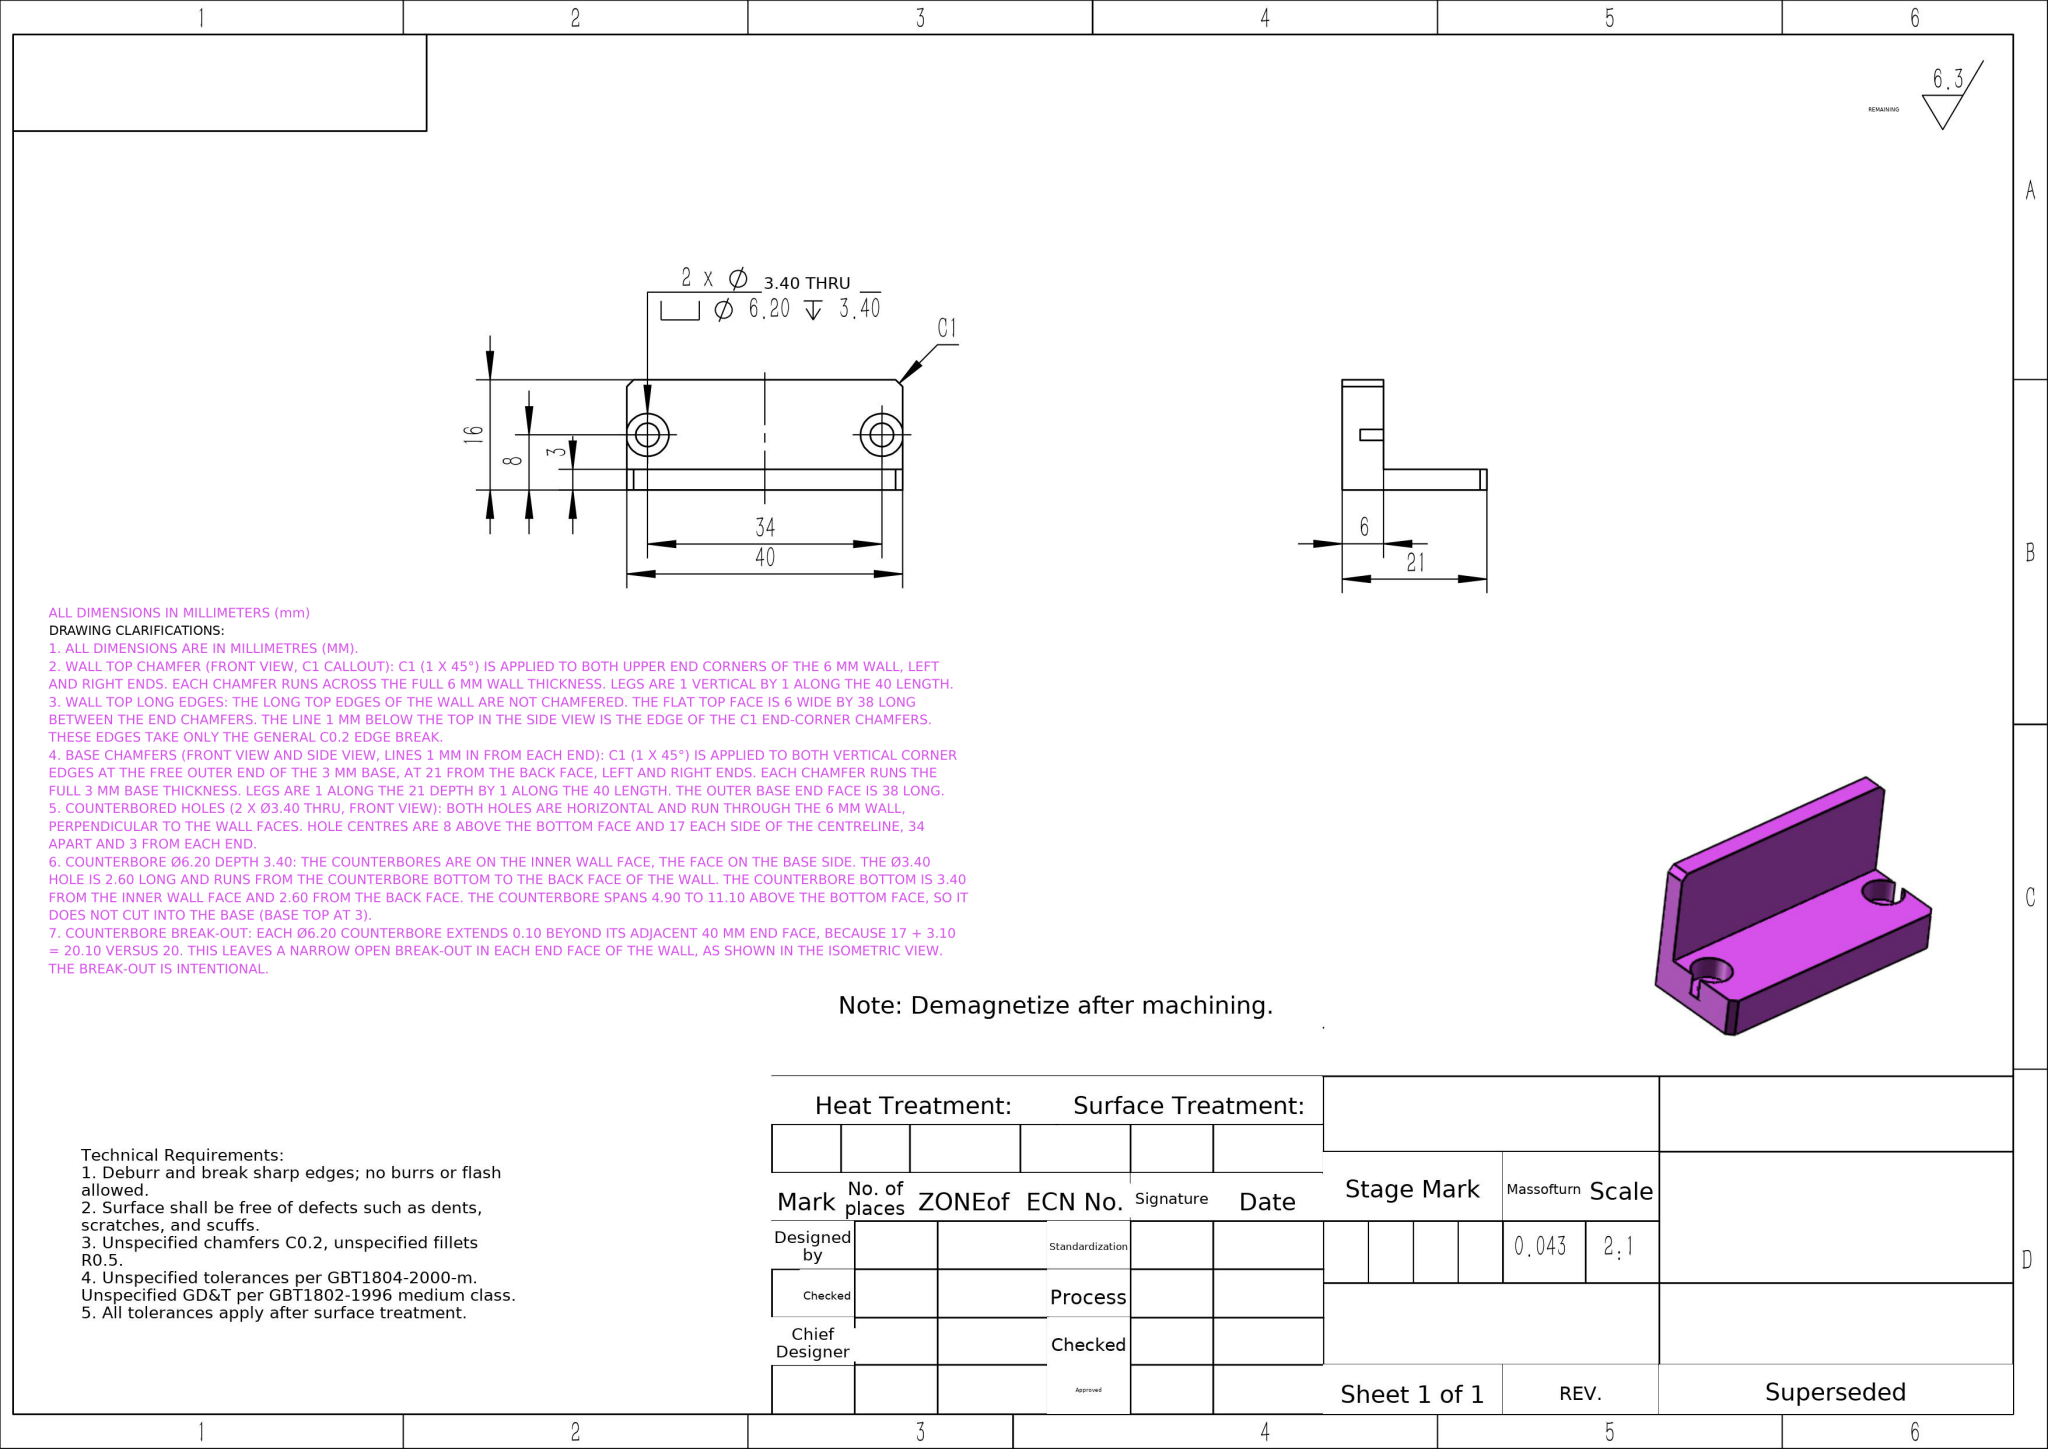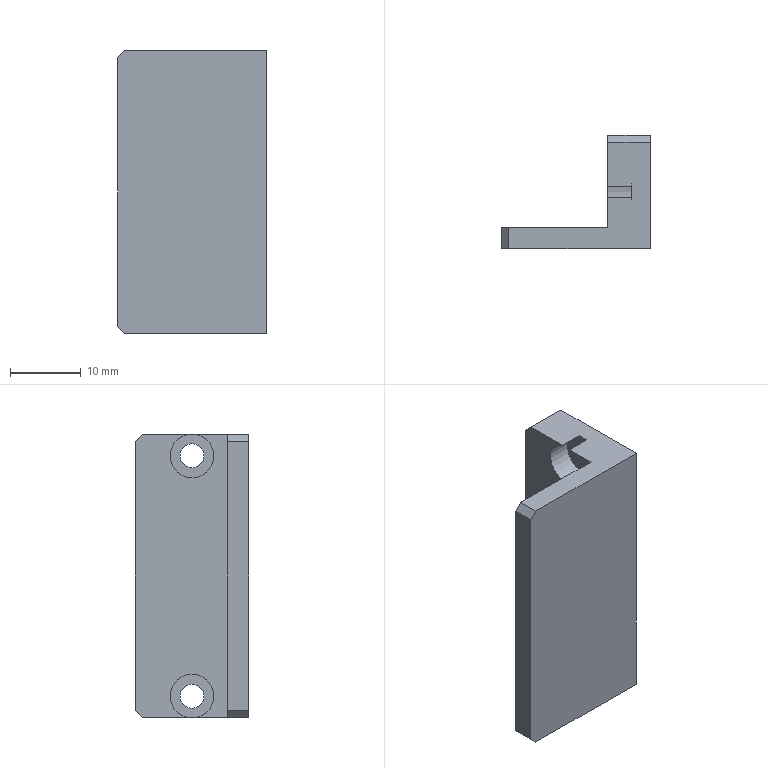Part | NX | mm | V-Notched Two-Bore Vertical Block | 1 solid | 21 faces | box 21 x 16 x 40 mm | volume 5379 mm3 | plane 14 | cylinder 7 | commonest cylinder face diameters 3.4 x4 6.2 x3
STEP:
#1=COLOUR_RGB('',0.6471,0.6196,0.5882);
#2=FILL_AREA_STYLE_COLOUR('',#1);
#3=FILL_AREA_STYLE('',(#2));
#4=SURFACE_STYLE_FILL_AREA(#3);
#5=SURFACE_SIDE_STYLE('',(#4));
#6=SURFACE_STYLE_USAGE(.BOTH.,#5);
#7=PRESENTATION_STYLE_ASSIGNMENT((#6));
#8=CARTESIAN_POINT('',(-2.6,-8.,-13.9));
#9=VERTEX_POINT('',#8);
#10=CARTESIAN_POINT('',(-2.6,-7.219,-20.));
#11=VERTEX_POINT('',#10);
#12=CARTESIAN_POINT('',(-2.6,-8.,-17.));
#13=DIRECTION('',(-1.,0.,0.));
#14=DIRECTION('',(0.,0.,1.));
#15=AXIS2_PLACEMENT_3D('',#12,#13,#14);
#16=CIRCLE('',#15,3.1);
#17=EDGE_CURVE('',#9,#11,#16,.T.);
#18=ORIENTED_EDGE('',*,*,#17,.F.);
#19=CARTESIAN_POINT('',(-6.,-8.,-13.9));
#20=VERTEX_POINT('',#19);
#21=CARTESIAN_POINT('',(-6.,-8.,-13.9));
#22=DIRECTION('',(-1.,0.,0.));
#23=VECTOR('',#22,1000.);
#24=LINE('',#21,#23);
#25=EDGE_CURVE('',#9,#20,#24,.T.);
#26=ORIENTED_EDGE('',*,*,#25,.T.);
#27=CARTESIAN_POINT('',(-6.,-7.219,-20.));
#28=VERTEX_POINT('',#27);
#29=CARTESIAN_POINT('',(-6.,-8.,-17.));
#30=DIRECTION('',(-1.,0.,0.));
#31=DIRECTION('',(0.,0.,1.));
#32=AXIS2_PLACEMENT_3D('',#29,#30,#31);
#33=CIRCLE('',#32,3.1);
#34=EDGE_CURVE('',#20,#28,#33,.T.);
#35=ORIENTED_EDGE('',*,*,#34,.T.);
#36=CARTESIAN_POINT('',(-6.,-7.219,-20.));
#37=DIRECTION('',(1.,0.,0.));
#38=VECTOR('',#37,1000.);
#39=LINE('',#36,#38);
#40=EDGE_CURVE('',#28,#11,#39,.T.);
#41=ORIENTED_EDGE('',*,*,#40,.T.);
#42=EDGE_LOOP('',(#18,#26,#35,#41));
#43=FACE_OUTER_BOUND('',#42,.T.);
#44=CARTESIAN_POINT('',(-6.,-8.,-17.));
#45=DIRECTION('',(-1.,0.,0.));
#46=DIRECTION('',(0.,0.,1.));
#47=AXIS2_PLACEMENT_3D('',#44,#45,#46);
#48=CYLINDRICAL_SURFACE('',#47,3.1);
#49=ADVANCED_FACE('',(#43),#48,.F.);
#50=CARTESIAN_POINT('',(0.,-8.,-18.7));
#51=VERTEX_POINT('',#50);
#52=CARTESIAN_POINT('',(0.,-8.,-15.3));
#53=VERTEX_POINT('',#52);
#54=CARTESIAN_POINT('',(0.,-8.,-17.));
#55=DIRECTION('',(-1.,-0.,0.));
#56=DIRECTION('',(0.,-1.,0.));
#57=AXIS2_PLACEMENT_3D('',#54,#55,#56);
#58=CIRCLE('',#57,1.7);
#59=EDGE_CURVE('',#51,#53,#58,.T.);
#60=ORIENTED_EDGE('',*,*,#59,.F.);
#61=CARTESIAN_POINT('',(-2.6,-8.,-18.7));
#62=VERTEX_POINT('',#61);
#63=CARTESIAN_POINT('',(-6.,-8.,-18.7));
#64=DIRECTION('',(-1.,0.,0.));
#65=VECTOR('',#64,1000.);
#66=LINE('',#63,#65);
#67=EDGE_CURVE('',#51,#62,#66,.T.);
#68=ORIENTED_EDGE('',*,*,#67,.T.);
#69=CARTESIAN_POINT('',(-2.6,-8.,-15.3));
#70=VERTEX_POINT('',#69);
#71=CARTESIAN_POINT('',(-2.6,-8.,-17.));
#72=DIRECTION('',(-1.,0.,0.));
#73=DIRECTION('',(0.,0.,1.));
#74=AXIS2_PLACEMENT_3D('',#71,#72,#73);
#75=CIRCLE('',#74,1.7);
#76=EDGE_CURVE('',#62,#70,#75,.T.);
#77=ORIENTED_EDGE('',*,*,#76,.T.);
#78=CARTESIAN_POINT('',(-6.,-8.,-15.3));
#79=DIRECTION('',(-1.,0.,0.));
#80=VECTOR('',#79,1000.);
#81=LINE('',#78,#80);
#82=EDGE_CURVE('',#53,#70,#81,.T.);
#83=ORIENTED_EDGE('',*,*,#82,.F.);
#84=EDGE_LOOP('',(#60,#68,#77,#83));
#85=FACE_OUTER_BOUND('',#84,.T.);
#86=CARTESIAN_POINT('',(-6.,-8.,-17.));
#87=DIRECTION('',(-1.,0.,0.));
#88=DIRECTION('',(0.,0.,1.));
#89=AXIS2_PLACEMENT_3D('',#86,#87,#88);
#90=CYLINDRICAL_SURFACE('',#89,1.7);
#91=ADVANCED_FACE('',(#85),#90,.F.);
#92=CARTESIAN_POINT('',(0.,-8.,15.3));
#93=VERTEX_POINT('',#92);
#94=CARTESIAN_POINT('',(0.,-8.,18.7));
#95=VERTEX_POINT('',#94);
#96=CARTESIAN_POINT('',(0.,-8.,17.));
#97=DIRECTION('',(-1.,-0.,0.));
#98=DIRECTION('',(0.,-1.,0.));
#99=AXIS2_PLACEMENT_3D('',#96,#97,#98);
#100=CIRCLE('',#99,1.7);
#101=EDGE_CURVE('',#93,#95,#100,.T.);
#102=ORIENTED_EDGE('',*,*,#101,.F.);
#103=CARTESIAN_POINT('',(-2.6,-8.,15.3));
#104=VERTEX_POINT('',#103);
#105=CARTESIAN_POINT('',(-6.,-8.,15.3));
#106=DIRECTION('',(-1.,0.,0.));
#107=VECTOR('',#106,1000.);
#108=LINE('',#105,#107);
#109=EDGE_CURVE('',#93,#104,#108,.T.);
#110=ORIENTED_EDGE('',*,*,#109,.T.);
#111=CARTESIAN_POINT('',(-2.6,-8.,18.7));
#112=VERTEX_POINT('',#111);
#113=CARTESIAN_POINT('',(-2.6,-8.,17.));
#114=DIRECTION('',(-1.,0.,0.));
#115=DIRECTION('',(0.,0.,1.));
#116=AXIS2_PLACEMENT_3D('',#113,#114,#115);
#117=CIRCLE('',#116,1.7);
#118=EDGE_CURVE('',#104,#112,#117,.T.);
#119=ORIENTED_EDGE('',*,*,#118,.T.);
#120=CARTESIAN_POINT('',(-6.,-8.,18.7));
#121=DIRECTION('',(-1.,0.,0.));
#122=VECTOR('',#121,1000.);
#123=LINE('',#120,#122);
#124=EDGE_CURVE('',#95,#112,#123,.T.);
#125=ORIENTED_EDGE('',*,*,#124,.F.);
#126=EDGE_LOOP('',(#102,#110,#119,#125));
#127=FACE_OUTER_BOUND('',#126,.T.);
#128=CARTESIAN_POINT('',(-6.,-8.,17.));
#129=DIRECTION('',(-1.,0.,0.));
#130=DIRECTION('',(0.,0.,1.));
#131=AXIS2_PLACEMENT_3D('',#128,#129,#130);
#132=CYLINDRICAL_SURFACE('',#131,1.7);
#133=ADVANCED_FACE('',(#127),#132,.F.);
#134=CARTESIAN_POINT('',(-6.,0.,19.));
#135=VERTEX_POINT('',#134);
#136=CARTESIAN_POINT('',(-6.,0.,-19.));
#137=VERTEX_POINT('',#136);
#138=CARTESIAN_POINT('',(-6.,0.,20.));
#139=DIRECTION('',(0.,0.,-1.));
#140=VECTOR('',#139,1000.);
#141=LINE('',#138,#140);
#142=EDGE_CURVE('',#135,#137,#141,.T.);
#143=ORIENTED_EDGE('',*,*,#142,.T.);
#144=CARTESIAN_POINT('',(-6.,-1.,-20.));
#145=VERTEX_POINT('',#144);
#146=CARTESIAN_POINT('',(-6.,0.,-19.));
#147=DIRECTION('',(0.,-0.7071,-0.7071));
#148=VECTOR('',#147,1000.);
#149=LINE('',#146,#148);
#150=EDGE_CURVE('',#137,#145,#149,.T.);
#151=ORIENTED_EDGE('',*,*,#150,.T.);
#152=CARTESIAN_POINT('',(-6.,-13.,-20.));
#153=DIRECTION('',(0.,-1.,0.));
#154=VECTOR('',#153,1000.);
#155=LINE('',#152,#154);
#156=EDGE_CURVE('',#145,#28,#155,.T.);
#157=ORIENTED_EDGE('',*,*,#156,.T.);
#158=ORIENTED_EDGE('',*,*,#34,.F.);
#159=CARTESIAN_POINT('',(-6.,-8.781,-20.));
#160=VERTEX_POINT('',#159);
#161=CARTESIAN_POINT('',(-6.,-8.,-17.));
#162=DIRECTION('',(-1.,0.,0.));
#163=DIRECTION('',(0.,0.,1.));
#164=AXIS2_PLACEMENT_3D('',#161,#162,#163);
#165=CIRCLE('',#164,3.1);
#166=EDGE_CURVE('',#160,#20,#165,.T.);
#167=ORIENTED_EDGE('',*,*,#166,.F.);
#168=CARTESIAN_POINT('',(-6.,-13.,-20.));
#169=VERTEX_POINT('',#168);
#170=CARTESIAN_POINT('',(-6.,-13.,-20.));
#171=DIRECTION('',(0.,-1.,0.));
#172=VECTOR('',#171,1000.);
#173=LINE('',#170,#172);
#174=EDGE_CURVE('',#160,#169,#173,.T.);
#175=ORIENTED_EDGE('',*,*,#174,.T.);
#176=CARTESIAN_POINT('',(-6.,-13.,20.));
#177=VERTEX_POINT('',#176);
#178=CARTESIAN_POINT('',(-6.,-13.,20.));
#179=DIRECTION('',(0.,0.,-1.));
#180=VECTOR('',#179,1000.);
#181=LINE('',#178,#180);
#182=EDGE_CURVE('',#177,#169,#181,.T.);
#183=ORIENTED_EDGE('',*,*,#182,.F.);
#184=CARTESIAN_POINT('',(-6.,-8.781,20.));
#185=VERTEX_POINT('',#184);
#186=CARTESIAN_POINT('',(-6.,-13.,20.));
#187=DIRECTION('',(0.,-1.,0.));
#188=VECTOR('',#187,1000.);
#189=LINE('',#186,#188);
#190=EDGE_CURVE('',#185,#177,#189,.T.);
#191=ORIENTED_EDGE('',*,*,#190,.F.);
#192=CARTESIAN_POINT('',(-6.,-7.219,20.));
#193=VERTEX_POINT('',#192);
#194=CARTESIAN_POINT('',(-6.,-8.,17.));
#195=DIRECTION('',(-1.,0.,0.));
#196=DIRECTION('',(0.,0.,1.));
#197=AXIS2_PLACEMENT_3D('',#194,#195,#196);
#198=CIRCLE('',#197,3.1);
#199=EDGE_CURVE('',#193,#185,#198,.T.);
#200=ORIENTED_EDGE('',*,*,#199,.F.);
#201=CARTESIAN_POINT('',(-6.,-1.,20.));
#202=VERTEX_POINT('',#201);
#203=CARTESIAN_POINT('',(-6.,-13.,20.));
#204=DIRECTION('',(0.,-1.,0.));
#205=VECTOR('',#204,1000.);
#206=LINE('',#203,#205);
#207=EDGE_CURVE('',#202,#193,#206,.T.);
#208=ORIENTED_EDGE('',*,*,#207,.F.);
#209=CARTESIAN_POINT('',(-6.,-1.,20.));
#210=DIRECTION('',(0.,0.7071,-0.7071));
#211=VECTOR('',#210,1000.);
#212=LINE('',#209,#211);
#213=EDGE_CURVE('',#202,#135,#212,.T.);
#214=ORIENTED_EDGE('',*,*,#213,.T.);
#215=EDGE_LOOP('',(#143,#151,#157,#158,#167,#175,#183,#191,#200,#208,#214));
#216=FACE_OUTER_BOUND('',#215,.T.);
#217=CARTESIAN_POINT('',(-6.,-13.,20.));
#218=DIRECTION('',(1.,0.,0.));
#219=DIRECTION('',(0.,0.,-1.));
#220=AXIS2_PLACEMENT_3D('',#217,#218,#219);
#221=PLANE('',#220);
#222=ADVANCED_FACE('',(#216),#221,.F.);
#223=CARTESIAN_POINT('',(0.,0.,19.));
#224=VERTEX_POINT('',#223);
#225=CARTESIAN_POINT('',(0.,0.,-19.));
#226=VERTEX_POINT('',#225);
#227=CARTESIAN_POINT('',(0.,0.,20.));
#228=DIRECTION('',(0.,0.,-1.));
#229=VECTOR('',#228,1000.);
#230=LINE('',#227,#229);
#231=EDGE_CURVE('',#224,#226,#230,.T.);
#232=ORIENTED_EDGE('',*,*,#231,.T.);
#233=CARTESIAN_POINT('',(-6.,0.,-19.));
#234=DIRECTION('',(-1.,0.,0.));
#235=VECTOR('',#234,1000.);
#236=LINE('',#233,#235);
#237=EDGE_CURVE('',#226,#137,#236,.T.);
#238=ORIENTED_EDGE('',*,*,#237,.T.);
#239=ORIENTED_EDGE('',*,*,#142,.F.);
#240=CARTESIAN_POINT('',(-6.,0.,19.));
#241=DIRECTION('',(1.,0.,0.));
#242=VECTOR('',#241,1000.);
#243=LINE('',#240,#242);
#244=EDGE_CURVE('',#135,#224,#243,.T.);
#245=ORIENTED_EDGE('',*,*,#244,.T.);
#246=EDGE_LOOP('',(#232,#238,#239,#245));
#247=FACE_OUTER_BOUND('',#246,.T.);
#248=CARTESIAN_POINT('',(-6.,0.,20.));
#249=DIRECTION('',(0.,-1.,0.));
#250=DIRECTION('',(0.,0.,-1.));
#251=AXIS2_PLACEMENT_3D('',#248,#249,#250);
#252=PLANE('',#251);
#253=ADVANCED_FACE('',(#247),#252,.F.);
#254=CARTESIAN_POINT('',(-20.,-13.,-20.));
#255=VERTEX_POINT('',#254);
#256=CARTESIAN_POINT('',(-21.,-13.,-20.));
#257=DIRECTION('',(-1.,0.,0.));
#258=VECTOR('',#257,1000.);
#259=LINE('',#256,#258);
#260=EDGE_CURVE('',#169,#255,#259,.T.);
#261=ORIENTED_EDGE('',*,*,#260,.T.);
#262=CARTESIAN_POINT('',(-21.,-13.,-19.));
#263=VERTEX_POINT('',#262);
#264=CARTESIAN_POINT('',(-21.,-13.,-19.));
#265=DIRECTION('',(-0.7071,0.,0.7071));
#266=VECTOR('',#265,1000.);
#267=LINE('',#264,#266);
#268=EDGE_CURVE('',#255,#263,#267,.T.);
#269=ORIENTED_EDGE('',*,*,#268,.T.);
#270=CARTESIAN_POINT('',(-21.,-13.,19.));
#271=VERTEX_POINT('',#270);
#272=CARTESIAN_POINT('',(-21.,-13.,20.));
#273=DIRECTION('',(0.,0.,-1.));
#274=VECTOR('',#273,1000.);
#275=LINE('',#272,#274);
#276=EDGE_CURVE('',#271,#263,#275,.T.);
#277=ORIENTED_EDGE('',*,*,#276,.F.);
#278=CARTESIAN_POINT('',(-20.,-13.,20.));
#279=VERTEX_POINT('',#278);
#280=CARTESIAN_POINT('',(-20.,-13.,20.));
#281=DIRECTION('',(0.7071,0.,0.7071));
#282=VECTOR('',#281,1000.);
#283=LINE('',#280,#282);
#284=EDGE_CURVE('',#271,#279,#283,.T.);
#285=ORIENTED_EDGE('',*,*,#284,.T.);
#286=CARTESIAN_POINT('',(-21.,-13.,20.));
#287=DIRECTION('',(-1.,0.,0.));
#288=VECTOR('',#287,1000.);
#289=LINE('',#286,#288);
#290=EDGE_CURVE('',#177,#279,#289,.T.);
#291=ORIENTED_EDGE('',*,*,#290,.F.);
#292=ORIENTED_EDGE('',*,*,#182,.T.);
#293=EDGE_LOOP('',(#261,#269,#277,#285,#291,#292));
#294=FACE_OUTER_BOUND('',#293,.T.);
#295=CARTESIAN_POINT('',(-21.,-13.,20.));
#296=DIRECTION('',(0.,-1.,0.));
#297=DIRECTION('',(0.,0.,-1.));
#298=AXIS2_PLACEMENT_3D('',#295,#296,#297);
#299=PLANE('',#298);
#300=ADVANCED_FACE('',(#294),#299,.F.);
#301=ORIENTED_EDGE('',*,*,#276,.T.);
#302=CARTESIAN_POINT('',(-21.,-16.,-19.));
#303=VERTEX_POINT('',#302);
#304=CARTESIAN_POINT('',(-21.,-16.,-19.));
#305=DIRECTION('',(0.,-1.,0.));
#306=VECTOR('',#305,1000.);
#307=LINE('',#304,#306);
#308=EDGE_CURVE('',#263,#303,#307,.T.);
#309=ORIENTED_EDGE('',*,*,#308,.T.);
#310=CARTESIAN_POINT('',(-21.,-16.,19.));
#311=VERTEX_POINT('',#310);
#312=CARTESIAN_POINT('',(-21.,-16.,20.));
#313=DIRECTION('',(0.,0.,-1.));
#314=VECTOR('',#313,1000.);
#315=LINE('',#312,#314);
#316=EDGE_CURVE('',#311,#303,#315,.T.);
#317=ORIENTED_EDGE('',*,*,#316,.F.);
#318=CARTESIAN_POINT('',(-21.,-16.,19.));
#319=DIRECTION('',(-0.,1.,0.));
#320=VECTOR('',#319,1000.);
#321=LINE('',#318,#320);
#322=EDGE_CURVE('',#311,#271,#321,.T.);
#323=ORIENTED_EDGE('',*,*,#322,.T.);
#324=EDGE_LOOP('',(#301,#309,#317,#323));
#325=FACE_OUTER_BOUND('',#324,.T.);
#326=CARTESIAN_POINT('',(-21.,-16.,20.));
#327=DIRECTION('',(1.,0.,0.));
#328=DIRECTION('',(-0.,1.,0.));
#329=AXIS2_PLACEMENT_3D('',#326,#327,#328);
#330=PLANE('',#329);
#331=ADVANCED_FACE('',(#325),#330,.F.);
#332=ORIENTED_EDGE('',*,*,#316,.T.);
#333=CARTESIAN_POINT('',(-20.,-16.,-20.));
#334=VERTEX_POINT('',#333);
#335=CARTESIAN_POINT('',(-21.,-16.,-19.));
#336=DIRECTION('',(0.7071,0.,-0.7071));
#337=VECTOR('',#336,1000.);
#338=LINE('',#335,#337);
#339=EDGE_CURVE('',#303,#334,#338,.T.);
#340=ORIENTED_EDGE('',*,*,#339,.T.);
#341=CARTESIAN_POINT('',(0.,-16.,-20.));
#342=VERTEX_POINT('',#341);
#343=CARTESIAN_POINT('',(0.,-16.,-20.));
#344=DIRECTION('',(1.,0.,0.));
#345=VECTOR('',#344,1000.);
#346=LINE('',#343,#345);
#347=EDGE_CURVE('',#334,#342,#346,.T.);
#348=ORIENTED_EDGE('',*,*,#347,.T.);
#349=CARTESIAN_POINT('',(0.,-16.,20.));
#350=VERTEX_POINT('',#349);
#351=CARTESIAN_POINT('',(0.,-16.,20.));
#352=DIRECTION('',(0.,0.,-1.));
#353=VECTOR('',#352,1000.);
#354=LINE('',#351,#353);
#355=EDGE_CURVE('',#350,#342,#354,.T.);
#356=ORIENTED_EDGE('',*,*,#355,.F.);
#357=CARTESIAN_POINT('',(-20.,-16.,20.));
#358=VERTEX_POINT('',#357);
#359=CARTESIAN_POINT('',(0.,-16.,20.));
#360=DIRECTION('',(1.,0.,0.));
#361=VECTOR('',#360,1000.);
#362=LINE('',#359,#361);
#363=EDGE_CURVE('',#358,#350,#362,.T.);
#364=ORIENTED_EDGE('',*,*,#363,.F.);
#365=CARTESIAN_POINT('',(-20.,-16.,20.));
#366=DIRECTION('',(-0.7071,-0.,-0.7071));
#367=VECTOR('',#366,1000.);
#368=LINE('',#365,#367);
#369=EDGE_CURVE('',#358,#311,#368,.T.);
#370=ORIENTED_EDGE('',*,*,#369,.T.);
#371=EDGE_LOOP('',(#332,#340,#348,#356,#364,#370));
#372=FACE_OUTER_BOUND('',#371,.T.);
#373=CARTESIAN_POINT('',(0.,-16.,20.));
#374=DIRECTION('',(-0.,1.,0.));
#375=DIRECTION('',(-1.,-0.,0.));
#376=AXIS2_PLACEMENT_3D('',#373,#374,#375);
#377=PLANE('',#376);
#378=ADVANCED_FACE('',(#372),#377,.F.);
#379=CARTESIAN_POINT('',(0.,-8.,-17.));
#380=DIRECTION('',(-1.,-0.,0.));
#381=DIRECTION('',(0.,-1.,0.));
#382=AXIS2_PLACEMENT_3D('',#379,#380,#381);
#383=CIRCLE('',#382,1.7);
#384=EDGE_CURVE('',#53,#51,#383,.T.);
#385=ORIENTED_EDGE('',*,*,#384,.T.);
#386=ORIENTED_EDGE('',*,*,#59,.T.);
#387=EDGE_LOOP('',(#385,#386));
#388=FACE_BOUND('',#387,.T.);
#389=CARTESIAN_POINT('',(0.,-8.,17.));
#390=DIRECTION('',(-1.,-0.,0.));
#391=DIRECTION('',(0.,-1.,0.));
#392=AXIS2_PLACEMENT_3D('',#389,#390,#391);
#393=CIRCLE('',#392,1.7);
#394=EDGE_CURVE('',#95,#93,#393,.T.);
#395=ORIENTED_EDGE('',*,*,#394,.T.);
#396=ORIENTED_EDGE('',*,*,#101,.T.);
#397=EDGE_LOOP('',(#395,#396));
#398=FACE_BOUND('',#397,.T.);
#399=CARTESIAN_POINT('',(0.,-1.,-20.));
#400=VERTEX_POINT('',#399);
#401=CARTESIAN_POINT('',(0.,0.,-20.));
#402=DIRECTION('',(-0.,1.,0.));
#403=VECTOR('',#402,1000.);
#404=LINE('',#401,#403);
#405=EDGE_CURVE('',#342,#400,#404,.T.);
#406=ORIENTED_EDGE('',*,*,#405,.T.);
#407=CARTESIAN_POINT('',(0.,0.,-19.));
#408=DIRECTION('',(-0.,0.7071,0.7071));
#409=VECTOR('',#408,1000.);
#410=LINE('',#407,#409);
#411=EDGE_CURVE('',#400,#226,#410,.T.);
#412=ORIENTED_EDGE('',*,*,#411,.T.);
#413=ORIENTED_EDGE('',*,*,#231,.F.);
#414=CARTESIAN_POINT('',(0.,-1.,20.));
#415=VERTEX_POINT('',#414);
#416=CARTESIAN_POINT('',(0.,-1.,20.));
#417=DIRECTION('',(0.,-0.7071,0.7071));
#418=VECTOR('',#417,1000.);
#419=LINE('',#416,#418);
#420=EDGE_CURVE('',#224,#415,#419,.T.);
#421=ORIENTED_EDGE('',*,*,#420,.T.);
#422=CARTESIAN_POINT('',(0.,0.,20.));
#423=DIRECTION('',(-0.,1.,0.));
#424=VECTOR('',#423,1000.);
#425=LINE('',#422,#424);
#426=EDGE_CURVE('',#350,#415,#425,.T.);
#427=ORIENTED_EDGE('',*,*,#426,.F.);
#428=ORIENTED_EDGE('',*,*,#355,.T.);
#429=EDGE_LOOP('',(#406,#412,#413,#421,#427,#428));
#430=FACE_OUTER_BOUND('',#429,.T.);
#431=CARTESIAN_POINT('',(0.,0.,20.));
#432=DIRECTION('',(-1.,-0.,0.));
#433=DIRECTION('',(0.,-1.,0.));
#434=AXIS2_PLACEMENT_3D('',#431,#432,#433);
#435=PLANE('',#434);
#436=ADVANCED_FACE('',(#388,#398,#430),#435,.F.);
#437=ORIENTED_EDGE('',*,*,#290,.T.);
#438=CARTESIAN_POINT('',(-20.,-0.,20.));
#439=DIRECTION('',(0.,-1.,0.));
#440=VECTOR('',#439,1000.);
#441=LINE('',#438,#440);
#442=EDGE_CURVE('',#279,#358,#441,.T.);
#443=ORIENTED_EDGE('',*,*,#442,.T.);
#444=ORIENTED_EDGE('',*,*,#363,.T.);
#445=ORIENTED_EDGE('',*,*,#426,.T.);
#446=CARTESIAN_POINT('',(0.,-1.,20.));
#447=DIRECTION('',(-1.,0.,0.));
#448=VECTOR('',#447,1000.);
#449=LINE('',#446,#448);
#450=EDGE_CURVE('',#415,#202,#449,.T.);
#451=ORIENTED_EDGE('',*,*,#450,.T.);
#452=ORIENTED_EDGE('',*,*,#207,.T.);
#453=CARTESIAN_POINT('',(-2.6,-7.219,20.));
#454=VERTEX_POINT('',#453);
#455=CARTESIAN_POINT('',(-6.,-7.219,20.));
#456=DIRECTION('',(1.,0.,0.));
#457=VECTOR('',#456,1000.);
#458=LINE('',#455,#457);
#459=EDGE_CURVE('',#193,#454,#458,.T.);
#460=ORIENTED_EDGE('',*,*,#459,.T.);
#461=CARTESIAN_POINT('',(-2.6,-8.781,20.));
#462=VERTEX_POINT('',#461);
#463=CARTESIAN_POINT('',(-2.6,0.,20.));
#464=DIRECTION('',(0.,-1.,0.));
#465=VECTOR('',#464,1000.);
#466=LINE('',#463,#465);
#467=EDGE_CURVE('',#454,#462,#466,.T.);
#468=ORIENTED_EDGE('',*,*,#467,.T.);
#469=CARTESIAN_POINT('',(-6.,-8.781,20.));
#470=DIRECTION('',(-1.,0.,0.));
#471=VECTOR('',#470,1000.);
#472=LINE('',#469,#471);
#473=EDGE_CURVE('',#462,#185,#472,.T.);
#474=ORIENTED_EDGE('',*,*,#473,.T.);
#475=ORIENTED_EDGE('',*,*,#190,.T.);
#476=EDGE_LOOP('',(#437,#443,#444,#445,#451,#452,#460,#468,#474,#475));
#477=FACE_OUTER_BOUND('',#476,.T.);
#478=CARTESIAN_POINT('',(0.,0.,20.));
#479=DIRECTION('',(0.,0.,-1.));
#480=DIRECTION('',(-1.,0.,0.));
#481=AXIS2_PLACEMENT_3D('',#478,#479,#480);
#482=PLANE('',#481);
#483=ADVANCED_FACE('',(#477),#482,.F.);
#484=ORIENTED_EDGE('',*,*,#347,.F.);
#485=CARTESIAN_POINT('',(-20.,-13.,-20.));
#486=DIRECTION('',(-0.,1.,0.));
#487=VECTOR('',#486,1000.);
#488=LINE('',#485,#487);
#489=EDGE_CURVE('',#334,#255,#488,.T.);
#490=ORIENTED_EDGE('',*,*,#489,.T.);
#491=ORIENTED_EDGE('',*,*,#260,.F.);
#492=ORIENTED_EDGE('',*,*,#174,.F.);
#493=CARTESIAN_POINT('',(-2.6,-8.781,-20.));
#494=VERTEX_POINT('',#493);
#495=CARTESIAN_POINT('',(-6.,-8.781,-20.));
#496=DIRECTION('',(-1.,0.,0.));
#497=VECTOR('',#496,1000.);
#498=LINE('',#495,#497);
#499=EDGE_CURVE('',#494,#160,#498,.T.);
#500=ORIENTED_EDGE('',*,*,#499,.F.);
#501=CARTESIAN_POINT('',(-2.6,0.,-20.));
#502=DIRECTION('',(0.,-1.,0.));
#503=VECTOR('',#502,1000.);
#504=LINE('',#501,#503);
#505=EDGE_CURVE('',#11,#494,#504,.T.);
#506=ORIENTED_EDGE('',*,*,#505,.F.);
#507=ORIENTED_EDGE('',*,*,#40,.F.);
#508=ORIENTED_EDGE('',*,*,#156,.F.);
#509=CARTESIAN_POINT('',(0.,-1.,-20.));
#510=DIRECTION('',(1.,0.,0.));
#511=VECTOR('',#510,1000.);
#512=LINE('',#509,#511);
#513=EDGE_CURVE('',#145,#400,#512,.T.);
#514=ORIENTED_EDGE('',*,*,#513,.T.);
#515=ORIENTED_EDGE('',*,*,#405,.F.);
#516=EDGE_LOOP('',(#484,#490,#491,#492,#500,#506,#507,#508,#514,#515));
#517=FACE_OUTER_BOUND('',#516,.T.);
#518=CARTESIAN_POINT('',(0.,0.,-20.));
#519=DIRECTION('',(0.,0.,-1.));
#520=DIRECTION('',(-1.,0.,0.));
#521=AXIS2_PLACEMENT_3D('',#518,#519,#520);
#522=PLANE('',#521);
#523=ADVANCED_FACE('',(#517),#522,.T.);
#524=CARTESIAN_POINT('',(-2.6,-8.,17.));
#525=DIRECTION('',(-1.,0.,0.));
#526=DIRECTION('',(0.,0.,1.));
#527=AXIS2_PLACEMENT_3D('',#524,#525,#526);
#528=CIRCLE('',#527,1.7);
#529=EDGE_CURVE('',#112,#104,#528,.T.);
#530=ORIENTED_EDGE('',*,*,#529,.F.);
#531=ORIENTED_EDGE('',*,*,#118,.F.);
#532=EDGE_LOOP('',(#530,#531));
#533=FACE_BOUND('',#532,.T.);
#534=CARTESIAN_POINT('',(-2.6,-8.,17.));
#535=DIRECTION('',(-1.,0.,0.));
#536=DIRECTION('',(0.,0.,1.));
#537=AXIS2_PLACEMENT_3D('',#534,#535,#536);
#538=CIRCLE('',#537,3.1);
#539=EDGE_CURVE('',#454,#462,#538,.T.);
#540=ORIENTED_EDGE('',*,*,#539,.T.);
#541=ORIENTED_EDGE('',*,*,#467,.F.);
#542=EDGE_LOOP('',(#540,#541));
#543=FACE_OUTER_BOUND('',#542,.T.);
#544=CARTESIAN_POINT('',(-2.6,-6.3,17.));
#545=DIRECTION('',(1.,0.,0.));
#546=DIRECTION('',(0.,0.,-1.));
#547=AXIS2_PLACEMENT_3D('',#544,#545,#546);
#548=PLANE('',#547);
#549=ADVANCED_FACE('',(#533,#543),#548,.F.);
#550=ORIENTED_EDGE('',*,*,#539,.F.);
#551=ORIENTED_EDGE('',*,*,#459,.F.);
#552=ORIENTED_EDGE('',*,*,#199,.T.);
#553=ORIENTED_EDGE('',*,*,#473,.F.);
#554=EDGE_LOOP('',(#550,#551,#552,#553));
#555=FACE_OUTER_BOUND('',#554,.T.);
#556=CARTESIAN_POINT('',(-6.,-8.,17.));
#557=DIRECTION('',(-1.,0.,0.));
#558=DIRECTION('',(0.,0.,1.));
#559=AXIS2_PLACEMENT_3D('',#556,#557,#558);
#560=CYLINDRICAL_SURFACE('',#559,3.1);
#561=ADVANCED_FACE('',(#555),#560,.F.);
#562=ORIENTED_EDGE('',*,*,#109,.F.);
#563=ORIENTED_EDGE('',*,*,#394,.F.);
#564=ORIENTED_EDGE('',*,*,#124,.T.);
#565=ORIENTED_EDGE('',*,*,#529,.T.);
#566=EDGE_LOOP('',(#562,#563,#564,#565));
#567=FACE_OUTER_BOUND('',#566,.T.);
#568=CARTESIAN_POINT('',(-6.,-8.,17.));
#569=DIRECTION('',(-1.,0.,0.));
#570=DIRECTION('',(0.,0.,1.));
#571=AXIS2_PLACEMENT_3D('',#568,#569,#570);
#572=CYLINDRICAL_SURFACE('',#571,1.7);
#573=ADVANCED_FACE('',(#567),#572,.F.);
#574=ORIENTED_EDGE('',*,*,#67,.F.);
#575=ORIENTED_EDGE('',*,*,#384,.F.);
#576=ORIENTED_EDGE('',*,*,#82,.T.);
#577=CARTESIAN_POINT('',(-2.6,-8.,-17.));
#578=DIRECTION('',(-1.,0.,0.));
#579=DIRECTION('',(0.,0.,1.));
#580=AXIS2_PLACEMENT_3D('',#577,#578,#579);
#581=CIRCLE('',#580,1.7);
#582=EDGE_CURVE('',#70,#62,#581,.T.);
#583=ORIENTED_EDGE('',*,*,#582,.T.);
#584=EDGE_LOOP('',(#574,#575,#576,#583));
#585=FACE_OUTER_BOUND('',#584,.T.);
#586=CARTESIAN_POINT('',(-6.,-8.,-17.));
#587=DIRECTION('',(-1.,0.,0.));
#588=DIRECTION('',(0.,0.,1.));
#589=AXIS2_PLACEMENT_3D('',#586,#587,#588);
#590=CYLINDRICAL_SURFACE('',#589,1.7);
#591=ADVANCED_FACE('',(#585),#590,.F.);
#592=ORIENTED_EDGE('',*,*,#505,.T.);
#593=CARTESIAN_POINT('',(-2.6,-8.,-17.));
#594=DIRECTION('',(-1.,0.,0.));
#595=DIRECTION('',(0.,0.,1.));
#596=AXIS2_PLACEMENT_3D('',#593,#594,#595);
#597=CIRCLE('',#596,3.1);
#598=EDGE_CURVE('',#494,#9,#597,.T.);
#599=ORIENTED_EDGE('',*,*,#598,.T.);
#600=ORIENTED_EDGE('',*,*,#17,.T.);
#601=EDGE_LOOP('',(#592,#599,#600));
#602=FACE_OUTER_BOUND('',#601,.T.);
#603=ORIENTED_EDGE('',*,*,#582,.F.);
#604=ORIENTED_EDGE('',*,*,#76,.F.);
#605=EDGE_LOOP('',(#603,#604));
#606=FACE_BOUND('',#605,.T.);
#607=CARTESIAN_POINT('',(-2.6,-6.3,-17.));
#608=DIRECTION('',(1.,0.,0.));
#609=DIRECTION('',(0.,0.,-1.));
#610=AXIS2_PLACEMENT_3D('',#607,#608,#609);
#611=PLANE('',#610);
#612=ADVANCED_FACE('',(#602,#606),#611,.F.);
#613=ORIENTED_EDGE('',*,*,#25,.F.);
#614=ORIENTED_EDGE('',*,*,#598,.F.);
#615=ORIENTED_EDGE('',*,*,#499,.T.);
#616=ORIENTED_EDGE('',*,*,#166,.T.);
#617=EDGE_LOOP('',(#613,#614,#615,#616));
#618=FACE_OUTER_BOUND('',#617,.T.);
#619=CARTESIAN_POINT('',(-6.,-8.,-17.));
#620=DIRECTION('',(-1.,0.,0.));
#621=DIRECTION('',(0.,0.,1.));
#622=AXIS2_PLACEMENT_3D('',#619,#620,#621);
#623=CYLINDRICAL_SURFACE('',#622,3.1);
#624=ADVANCED_FACE('',(#618),#623,.F.);
#625=ORIENTED_EDGE('',*,*,#268,.F.);
#626=ORIENTED_EDGE('',*,*,#489,.F.);
#627=ORIENTED_EDGE('',*,*,#339,.F.);
#628=ORIENTED_EDGE('',*,*,#308,.F.);
#629=EDGE_LOOP('',(#625,#626,#627,#628));
#630=FACE_OUTER_BOUND('',#629,.T.);
#631=CARTESIAN_POINT('',(-21.,-16.,-19.));
#632=DIRECTION('',(-0.7071,-0.,-0.7071));
#633=DIRECTION('',(-0.,1.,0.));
#634=AXIS2_PLACEMENT_3D('',#631,#632,#633);
#635=PLANE('',#634);
#636=ADVANCED_FACE('',(#630),#635,.T.);
#637=ORIENTED_EDGE('',*,*,#284,.F.);
#638=ORIENTED_EDGE('',*,*,#322,.F.);
#639=ORIENTED_EDGE('',*,*,#369,.F.);
#640=ORIENTED_EDGE('',*,*,#442,.F.);
#641=EDGE_LOOP('',(#637,#638,#639,#640));
#642=FACE_OUTER_BOUND('',#641,.T.);
#643=CARTESIAN_POINT('',(-20.,-0.,20.));
#644=DIRECTION('',(0.7071,0.,-0.7071));
#645=DIRECTION('',(0.,-1.,0.));
#646=AXIS2_PLACEMENT_3D('',#643,#644,#645);
#647=PLANE('',#646);
#648=ADVANCED_FACE('',(#642),#647,.F.);
#649=ORIENTED_EDGE('',*,*,#411,.F.);
#650=ORIENTED_EDGE('',*,*,#513,.F.);
#651=ORIENTED_EDGE('',*,*,#150,.F.);
#652=ORIENTED_EDGE('',*,*,#237,.F.);
#653=EDGE_LOOP('',(#649,#650,#651,#652));
#654=FACE_OUTER_BOUND('',#653,.T.);
#655=CARTESIAN_POINT('',(-6.,0.,-19.));
#656=DIRECTION('',(0.,0.7071,-0.7071));
#657=DIRECTION('',(1.,0.,0.));
#658=AXIS2_PLACEMENT_3D('',#655,#656,#657);
#659=PLANE('',#658);
#660=ADVANCED_FACE('',(#654),#659,.T.);
#661=ORIENTED_EDGE('',*,*,#420,.F.);
#662=ORIENTED_EDGE('',*,*,#244,.F.);
#663=ORIENTED_EDGE('',*,*,#213,.F.);
#664=ORIENTED_EDGE('',*,*,#450,.F.);
#665=EDGE_LOOP('',(#661,#662,#663,#664));
#666=FACE_OUTER_BOUND('',#665,.T.);
#667=CARTESIAN_POINT('',(0.,-1.,20.));
#668=DIRECTION('',(0.,-0.7071,-0.7071));
#669=DIRECTION('',(-1.,0.,0.));
#670=AXIS2_PLACEMENT_3D('',#667,#668,#669);
#671=PLANE('',#670);
#672=ADVANCED_FACE('',(#666),#671,.F.);
#673=CLOSED_SHELL('',(#49,#91,#133,#222,#253,#300,#331,#378,#436,#483,#523,#549,#561,#573,#591,#612,#624,#636,#648,#660,#672));
#674=MANIFOLD_SOLID_BREP('',#673);
#675=STYLED_ITEM('',(#7),#674);
#676=PRESENTATION_LAYER_ASSIGNMENT('','',(#675));
#677=COLOUR_RGB('',0.6471,0.6196,0.5882);
#678=FILL_AREA_STYLE_COLOUR('',#677);
#679=FILL_AREA_STYLE('',(#678));
#680=SURFACE_STYLE_FILL_AREA(#679);
#681=SURFACE_SIDE_STYLE('',(#680));
#682=SURFACE_STYLE_USAGE(.BOTH.,#681);
#683=PRESENTATION_STYLE_ASSIGNMENT((#682));
#684=CARTESIAN_POINT('',(0.,0.,0.));
#685=DIRECTION('',(0.,0.,1.));
#686=DIRECTION('',(1.,0.,0.));
#687=AXIS2_PLACEMENT_3D('',#684,#685,#686);
#688=(LENGTH_UNIT()NAMED_UNIT(*)SI_UNIT(.MILLI.,.METRE.));
#689=UNCERTAINTY_MEASURE_WITH_UNIT(LENGTH_MEASURE(0.00001),#688,'','');
#690=(NAMED_UNIT(*)PLANE_ANGLE_UNIT()SI_UNIT($,.RADIAN.));
#691=(NAMED_UNIT(*)SI_UNIT($,.STERADIAN.)SOLID_ANGLE_UNIT());
#692=(GEOMETRIC_REPRESENTATION_CONTEXT(3)GLOBAL_UNCERTAINTY_ASSIGNED_CONTEXT((#689))GLOBAL_UNIT_ASSIGNED_CONTEXT((#688,#690,#691))REPRESENTATION_CONTEXT('',''));
#693=ADVANCED_BREP_SHAPE_REPRESENTATION('',(#674,#687),#692);
#694=STYLED_ITEM('',(#683),#693);
#695=(LENGTH_UNIT()NAMED_UNIT(*)SI_UNIT(.MILLI.,.METRE.));
#696=UNCERTAINTY_MEASURE_WITH_UNIT(LENGTH_MEASURE(0.00001),#695,'','');
#697=(NAMED_UNIT(*)PLANE_ANGLE_UNIT()SI_UNIT($,.RADIAN.));
#698=(NAMED_UNIT(*)SI_UNIT($,.STERADIAN.)SOLID_ANGLE_UNIT());
#699=(GEOMETRIC_REPRESENTATION_CONTEXT(3)GLOBAL_UNCERTAINTY_ASSIGNED_CONTEXT((#696))GLOBAL_UNIT_ASSIGNED_CONTEXT((#695,#697,#698))REPRESENTATION_CONTEXT('',''));
#700=MECHANICAL_DESIGN_GEOMETRIC_PRESENTATION_REPRESENTATION('',(#694),#699);
#701=(LENGTH_UNIT()NAMED_UNIT(*)SI_UNIT(.MILLI.,.METRE.));
#702=UNCERTAINTY_MEASURE_WITH_UNIT(LENGTH_MEASURE(0.00001),#701,'','');
#703=(NAMED_UNIT(*)PLANE_ANGLE_UNIT()SI_UNIT($,.RADIAN.));
#704=(NAMED_UNIT(*)SI_UNIT($,.STERADIAN.)SOLID_ANGLE_UNIT());
#705=(GEOMETRIC_REPRESENTATION_CONTEXT(3)GLOBAL_UNCERTAINTY_ASSIGNED_CONTEXT((#702))GLOBAL_UNIT_ASSIGNED_CONTEXT((#701,#703,#704))REPRESENTATION_CONTEXT('',''));
#706=MECHANICAL_DESIGN_GEOMETRIC_PRESENTATION_REPRESENTATION('',(#675),#705);
#707=PRESENTATION_LAYER_ASSIGNMENT('','',(#694));